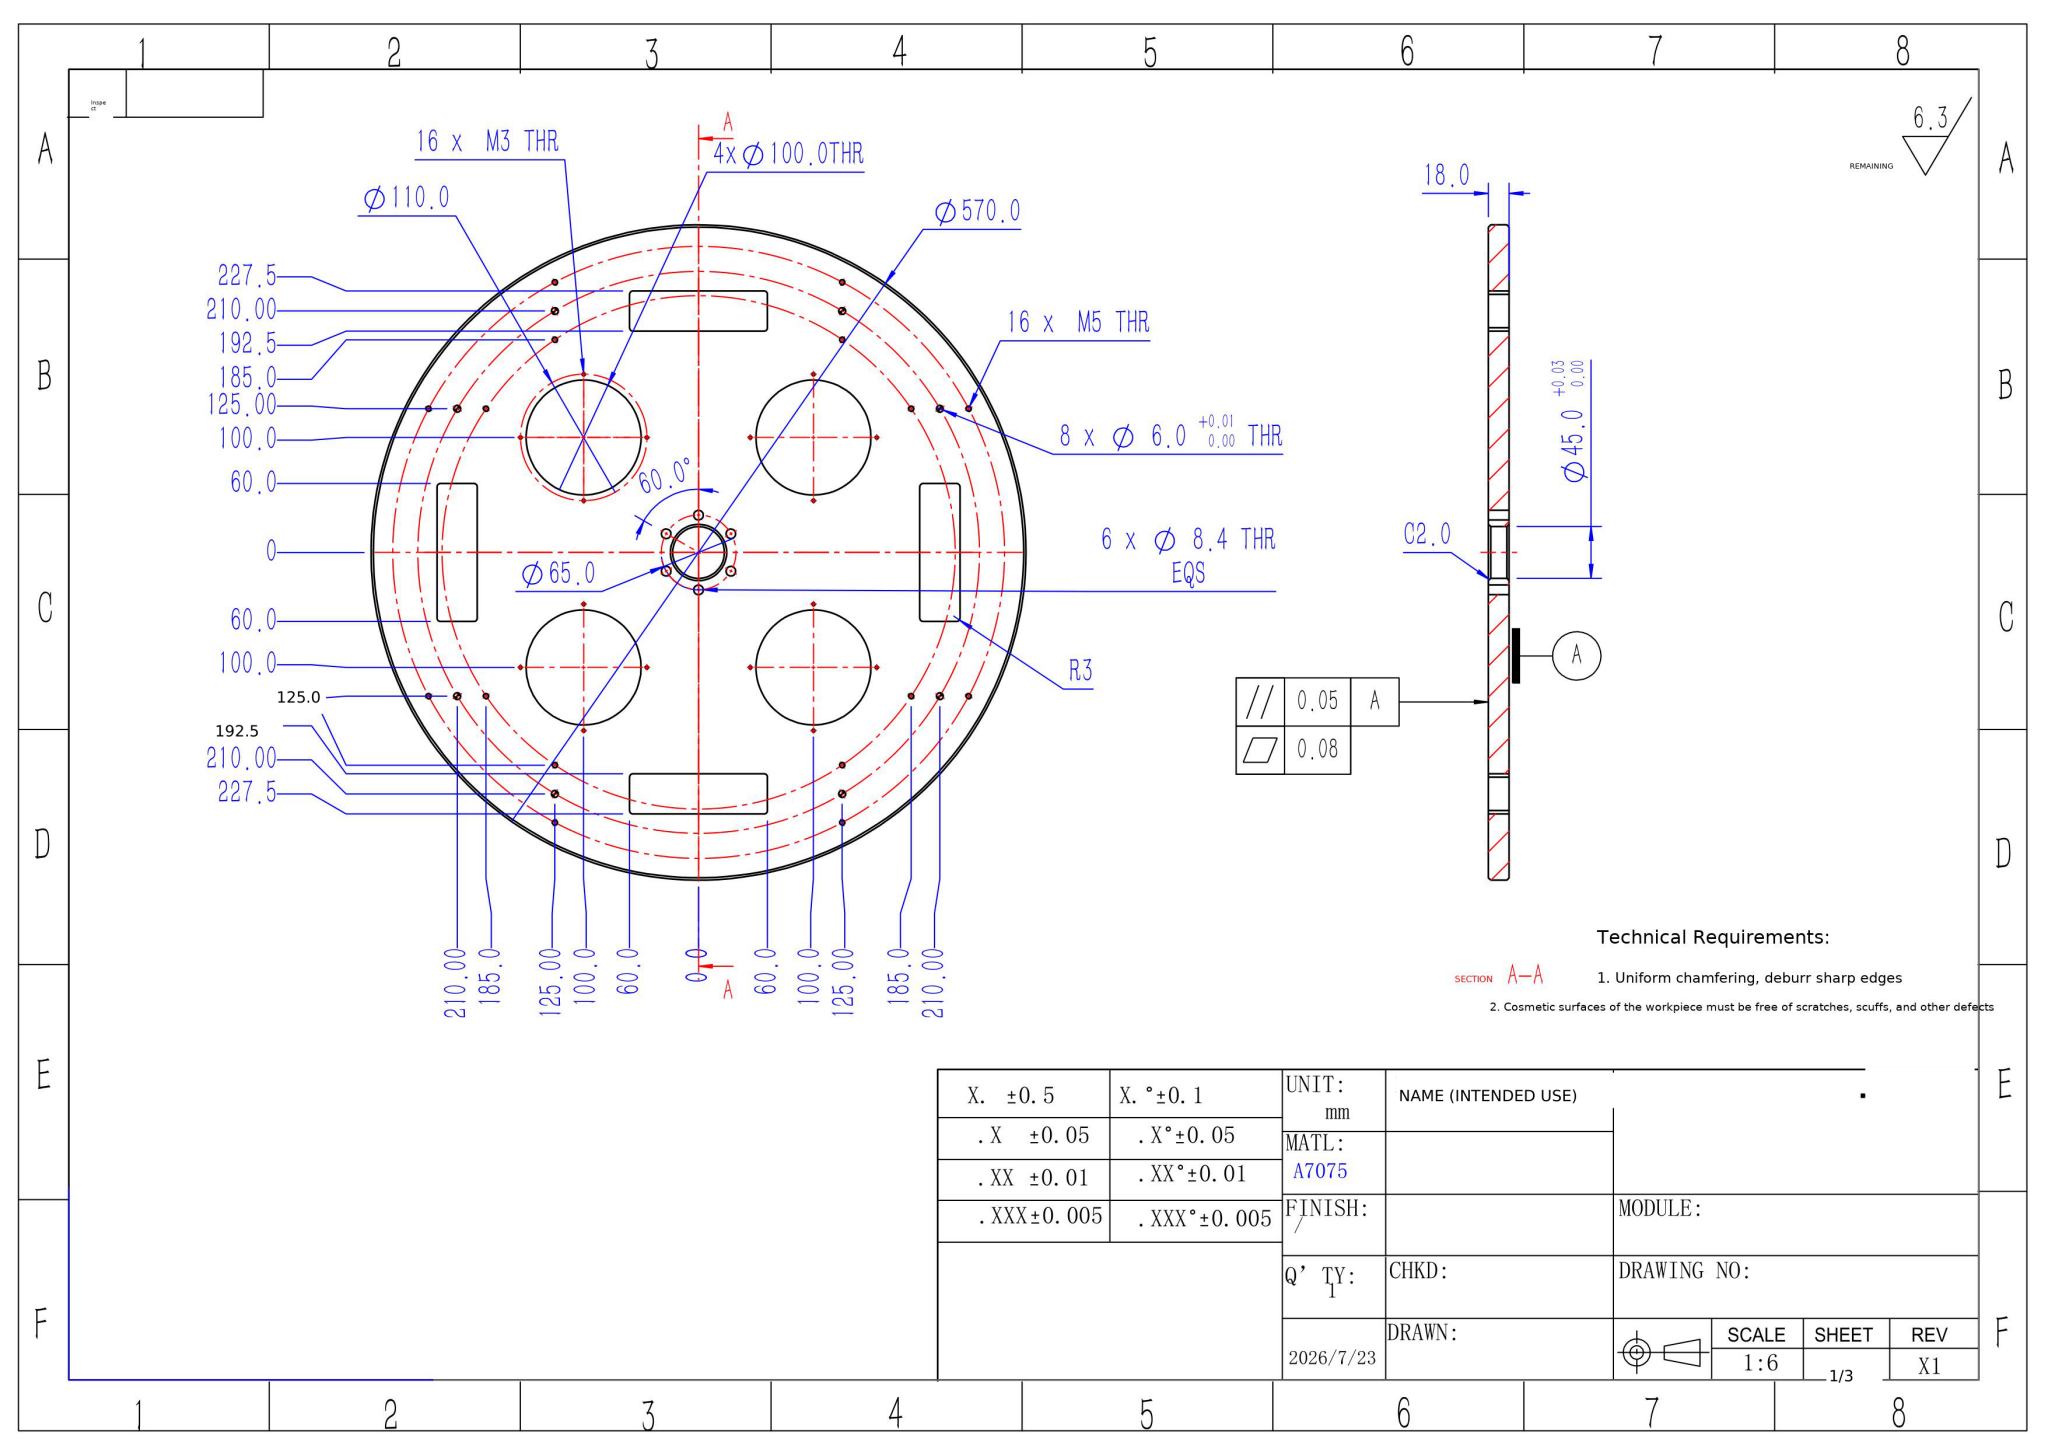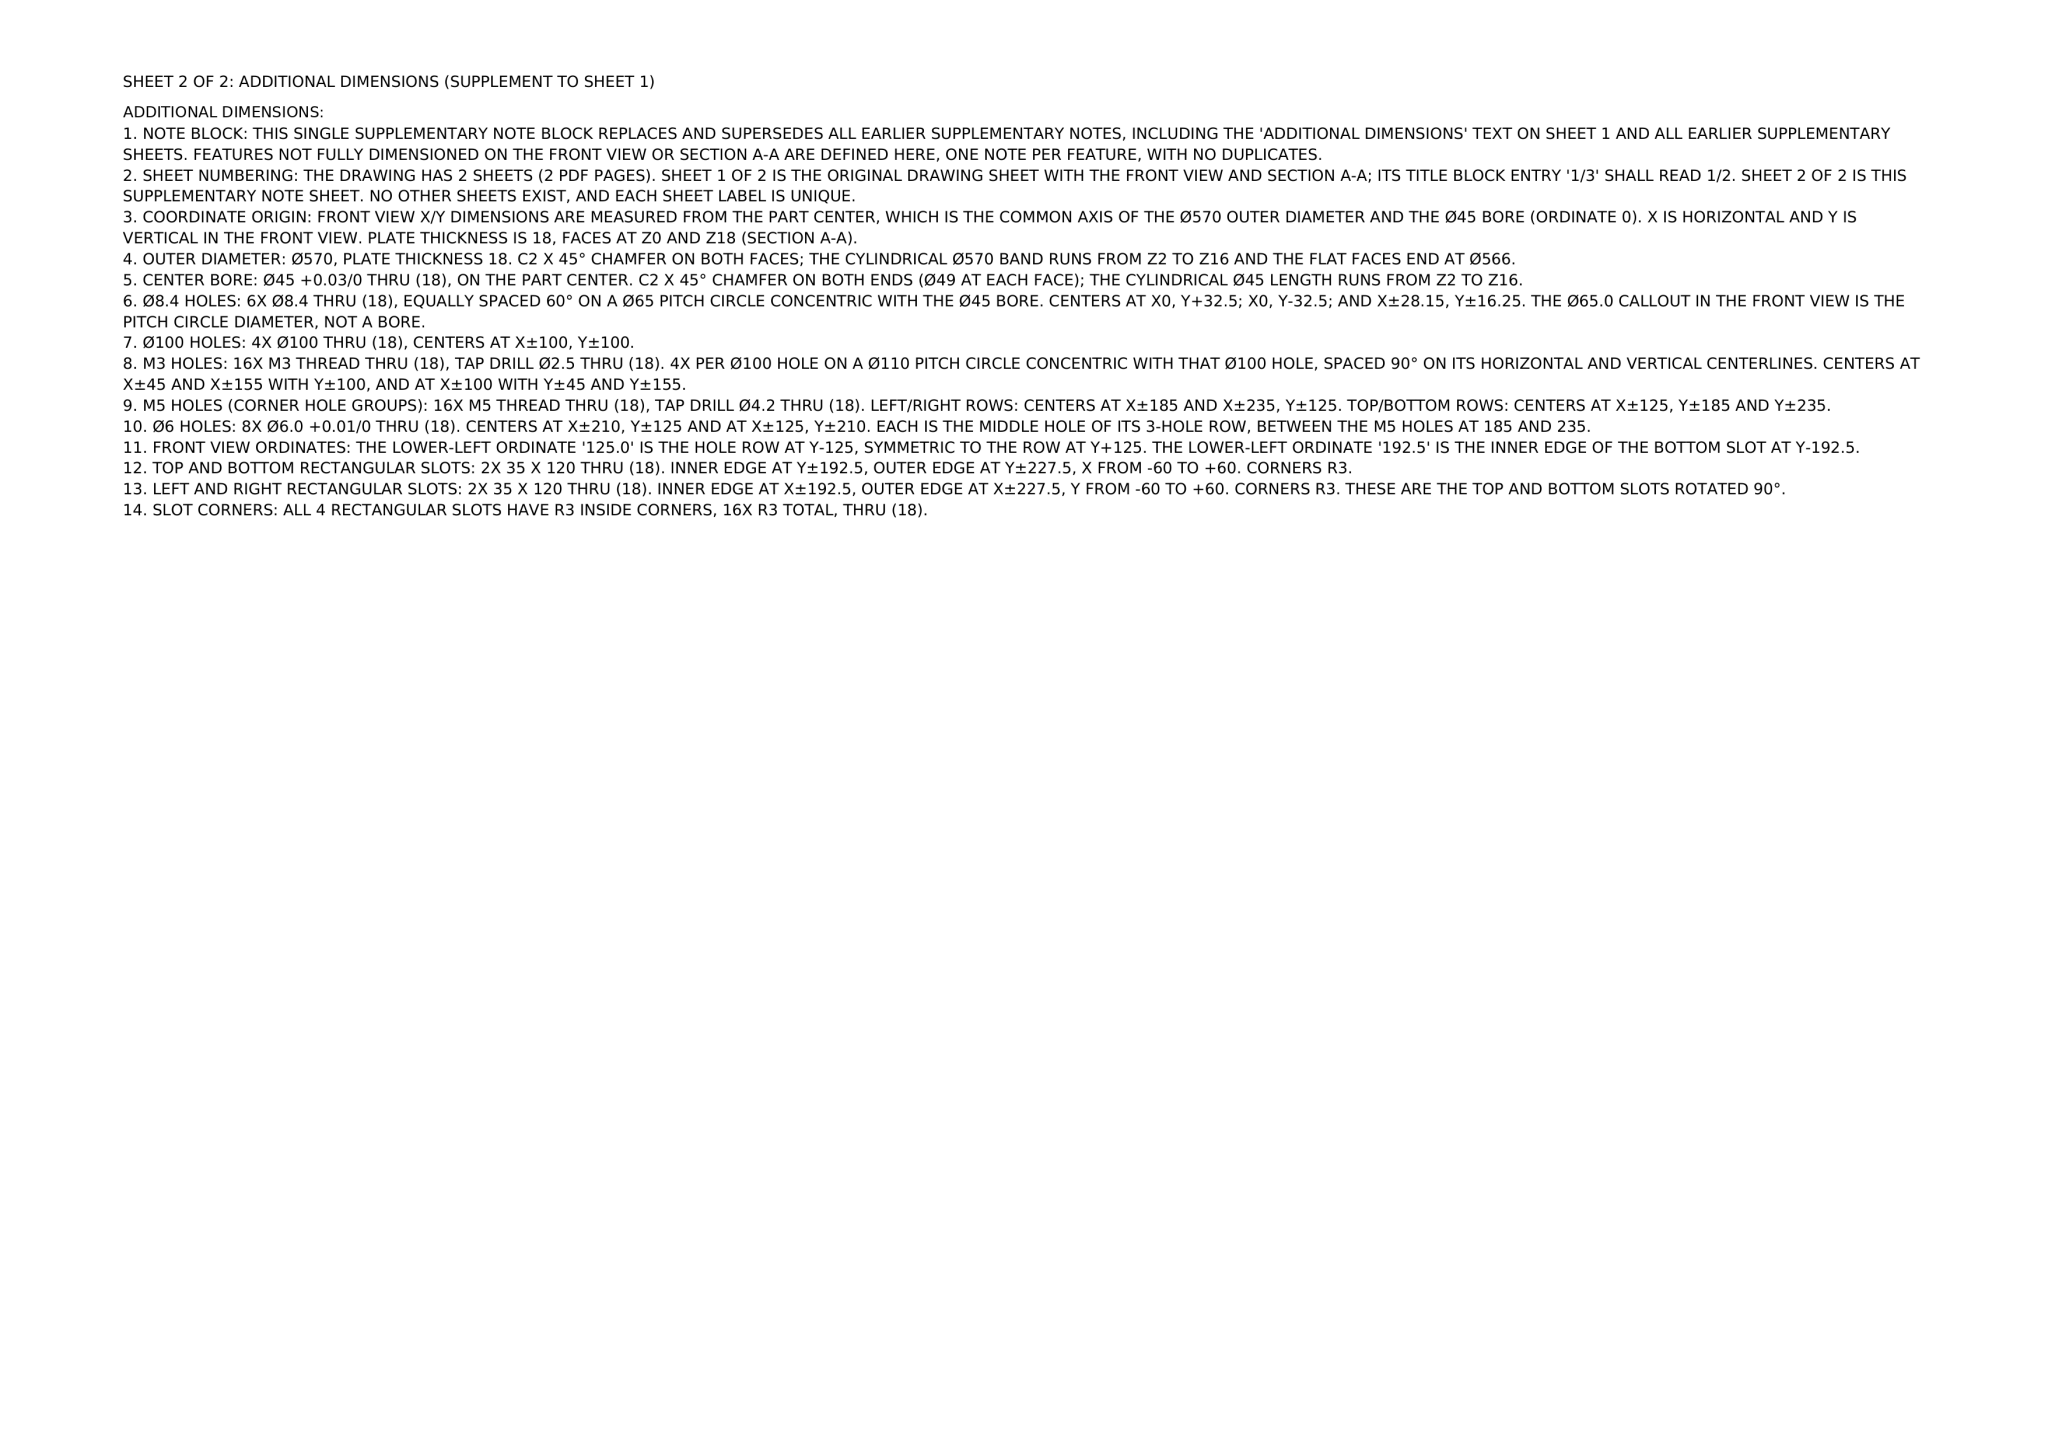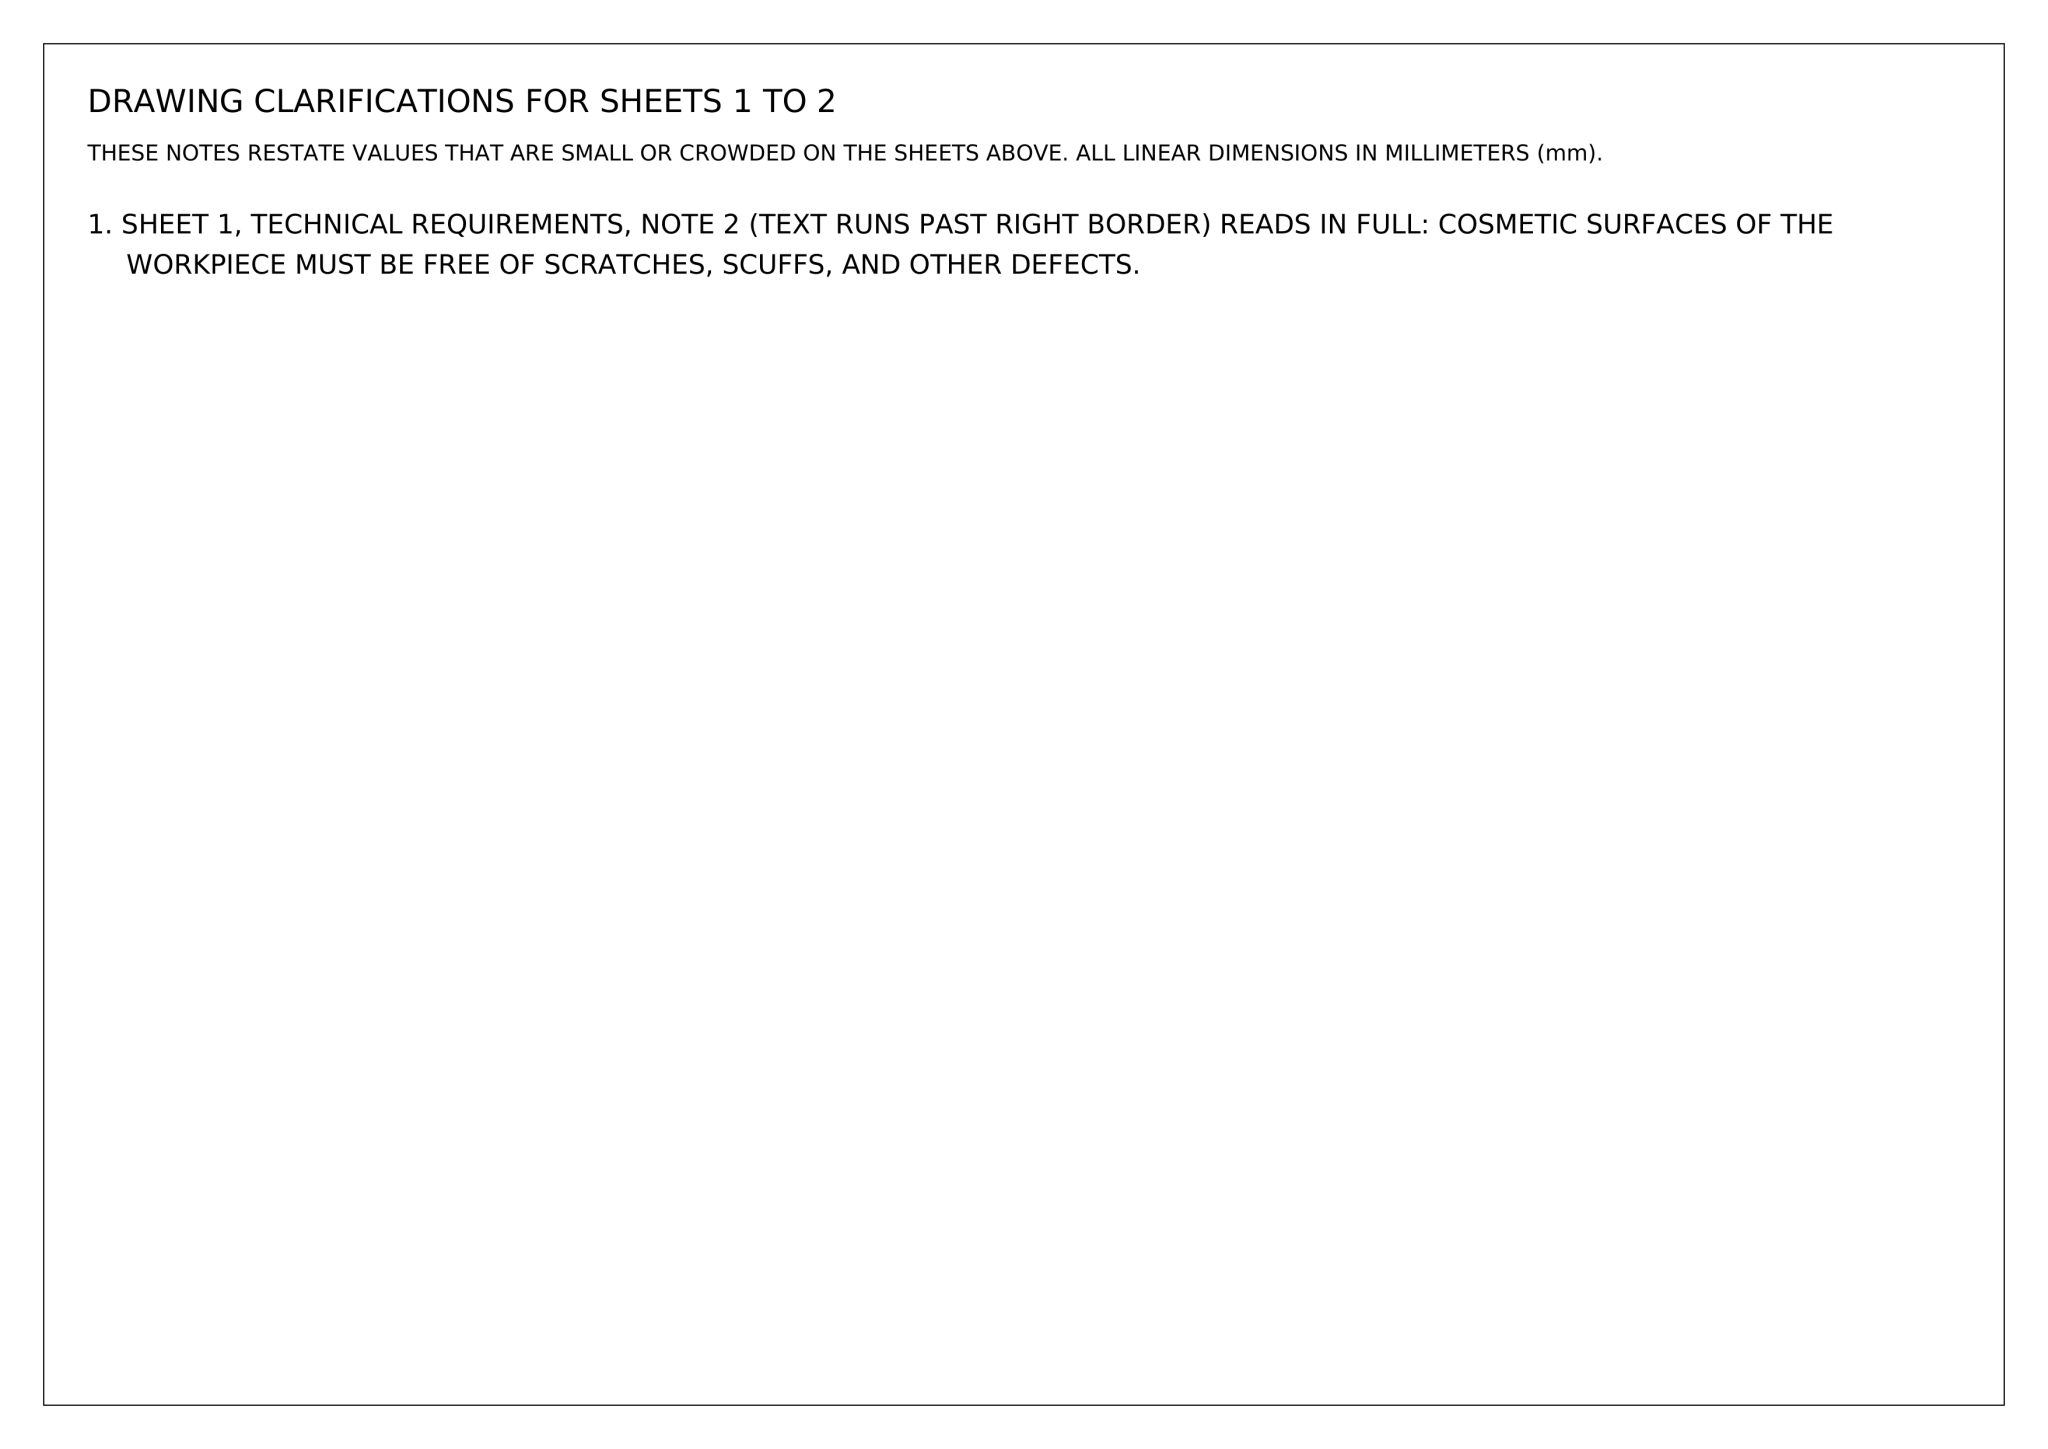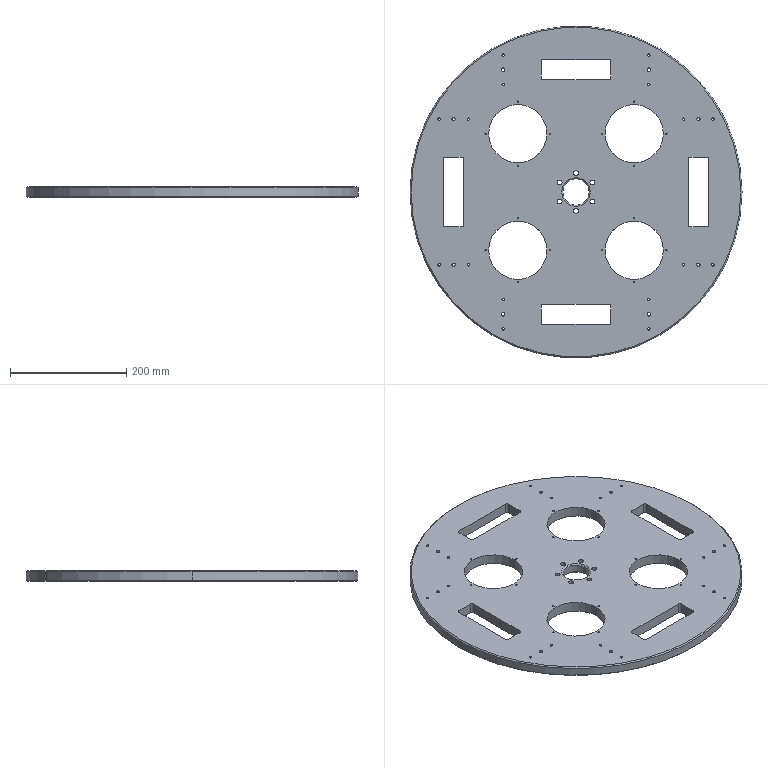Part | NX | mm | 1 solid | 146 faces | box 570 x 570 x 18 mm | volume 3674019 mm3 | cylinder 120 | plane 18 | cone 8 | commonest cylinder face diameters 2.5 x32 6 x32 4.2 x32 8.4 x12 100 x8 45 x2 570 x2